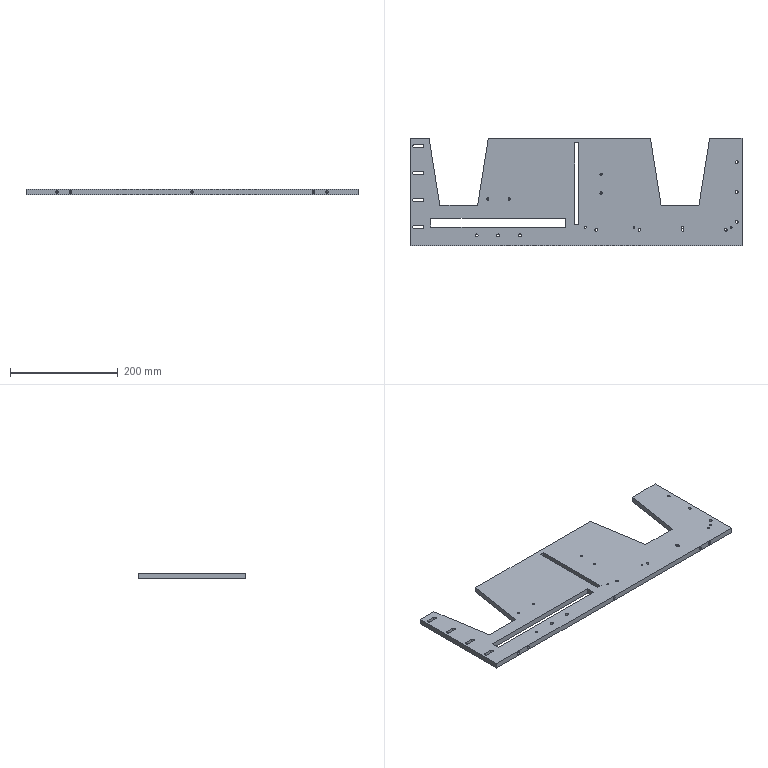Component | SolidWorks | P-SLJ-001-008-1 | 1 solid | 108 faces | box 615 x 200 x 10 mm | volume 942437 mm3 | cylinder 64 | plane 34 | cone 10 | commonest cylinder face diameters 5.5 x24 5 x18 3.3 x8 4.2 x8 10 x6 | material 45#
build123d program:
from build123d import *

# Parameters (mm, degrees)
SKETCH1_W                                            = 615
SKETCH1_H                                            = 200
EXTRUDE1_DEPTH                                       = 5
TAP_DRILL_FOR_M4X0_5_TAP1_D                          = 5.5
EXTRUDE2_DEPTH                                       = 324.506
M6_TAPPED_HOLE1_D                                    = 5
SKETCH9_W                                            = 8
SKETCH9_H                                            = 151
EXTRUDE3_DEPTH                                       = 324.506
EXTRUDE4_DEPTH                                       = 324.506
M5_TAPPED_HOLE1_2_D                                  = 4.2
HOLE_SIZE_ACCORDING_TO_TYPE_OF_HEX_SOCKE_D           = 5.5
HOLE_SIZE_ACCORDING_TO_TYPE_OF_HEX_SOCKE_CBORE_D     = 10
HOLE_SIZE_ACCORDING_TO_TYPE_OF_HEX_SOCKE_CBORE_DEPTH = 5.7
SKETCH16_W                                           = 250
SKETCH16_H                                           = 16
EXTRUDE5_DEPTH                                       = 324.506
M5_TAPPED_HOLE1_D                                    = 4.2
CHAMFER1_SIZE                                        = 2
CHAMFER1_SIZE2                                       = 5
M4_TAPPED_HOLE3_D                                    = 3.3
F_5_0_5_DIAMETER_HOLE1_D                             = 5
F_5_0_5_DIAMETER_HOLE1_DEPTH                         = 10
F_5_0_5_DIAMETER_HOLE1_TIP                           = 1.502
M6_TAPPED_HOLE2_D                                    = 5
M6_TAPPED_HOLE2_DEPTH                                = 17
M6_TAPPED_HOLE2_TIP                                  = 1.502


with BuildPart() as part:
    # Sketch1 → Extrude1 (new, symmetric)
    with BuildSketch(Plane.XY):
        Rectangle(SKETCH1_W, SKETCH1_H)
    extrude(amount=EXTRUDE1_DEPTH, both=True)

    # Tap Drill for M4X0.5 Tap1 (through all)
    with Locations(Plane.XY.offset(5)):
        with Locations((297.5, 55), (297.5, 0), (297.5, -55)):
            Hole(TAP_DRILL_FOR_M4X0_5_TAP1_D / 2)

    # Sketch5 → Extrude2 (cut, through all)
    with BuildSketch(Plane.XY.offset(5)):
        Polygon((137.904, 100), (247.5, 100), (227.702, -25), (157.702, -25), align=None)
        Polygon((-272.096, 100), (-162.5, 100), (-182.298, -25), (-252.298, -25), align=None)
    extrude(amount=-EXTRUDE2_DEPTH, mode=Mode.SUBTRACT)

    # M6 Tapped Hole1 (through all)
    with Locations(Plane.XY.offset(5)):
        with Locations((37.5, -70), (117.5, -70), (197.5, -70), (277.5, -70)):
            Hole(M6_TAPPED_HOLE1_D / 2)

    # Sketch9 → Extrude3 (cut, through all)
    with BuildSketch(Plane.XY.offset(5)):
        with Locations((1.5, 15.5)):
            Rectangle(SKETCH9_W, SKETCH9_H)
    extrude(amount=-EXTRUDE3_DEPTH, mode=Mode.SUBTRACT)

    # Sketch10 → Extrude4 (cut, through all)
    with BuildSketch(Plane.XY.offset(5)):
        with BuildLine():
            Line((-300, 87.75), (-285, 87.75))
            ThreePointArc((-285, 87.75), (-282.25, 85), (-285, 82.25))
            Line((-285, 82.25), (-300, 82.25))
            ThreePointArc((-300, 82.25), (-302.75, 85), (-300, 87.75))
        make_face()
        with BuildLine():
            Line((-300, 37.75), (-285, 37.75))
            ThreePointArc((-285, 37.75), (-282.25, 35), (-285, 32.25))
            Line((-285, 32.25), (-300, 32.25))
            ThreePointArc((-300, 32.25), (-302.75, 35), (-300, 37.75))
        make_face()
        with BuildLine():
            Line((-300, -12.25), (-285, -12.25))
            ThreePointArc((-285, -12.25), (-282.25, -15), (-285, -17.75))
            Line((-285, -17.75), (-300, -17.75))
            ThreePointArc((-300, -17.75), (-302.75, -15), (-300, -12.25))
        make_face()
        with BuildLine():
            Line((-300, -62.25), (-285, -62.25))
            ThreePointArc((-285, -62.25), (-282.25, -65), (-285, -67.75))
            Line((-285, -67.75), (-300, -67.75))
            ThreePointArc((-300, -67.75), (-302.75, -65), (-300, -62.25))
        make_face()
    extrude(amount=-EXTRUDE4_DEPTH, mode=Mode.SUBTRACT)

    # M5 Tapped Hole1_2 (through all)
    with Locations(Plane.XY.offset(5)):
        with Locations((-163.5, -13), (-123.5, -13)):
            Hole(M5_TAPPED_HOLE1_2_D / 2)

    # Hole Size_according to_Type of Hex Socke (through all)
    with Locations(Plane(origin=(0, 0, -5), x_dir=(-1, 0, 0), z_dir=(0, 0, -1))):
        with Locations((184, -80.5), (144, -80.5), (104, -80.5)):
            CounterBoreHole(HOLE_SIZE_ACCORDING_TO_TYPE_OF_HEX_SOCKE_D / 2, HOLE_SIZE_ACCORDING_TO_TYPE_OF_HEX_SOCKE_CBORE_D / 2, HOLE_SIZE_ACCORDING_TO_TYPE_OF_HEX_SOCKE_CBORE_DEPTH)

    # Sketch16 → Extrude5 (cut, through all)
    with BuildSketch(Plane.XY.offset(5)):
        with Locations((-144, -57)):
            Rectangle(SKETCH16_W, SKETCH16_H)
    extrude(amount=-EXTRUDE5_DEPTH, mode=Mode.SUBTRACT)

    # M5 Tapped Hole1 (through all)
    with Locations(Plane.XY.offset(5)):
        with Locations((46.5, 33), (46.5, -2)):
            Hole(M5_TAPPED_HOLE1_D / 2)

    # Chamfer1
    chamfer1_edges = [part.edges().sort_by_distance(p)[0] for p in [
        (-144, -65, -5),
    ]]
    chamfer1_side = [part.faces().sort_by_distance(p)[0] for p in [
        (-144, -65, 0),
    ]]
    chamfer(chamfer1_edges, length=CHAMFER1_SIZE, length2=CHAMFER1_SIZE2, reference=chamfer1_side[0])

    # M4 Tapped Hole3 (through all)
    with Locations(Plane(origin=(0, 0, -5), x_dir=(-1, 0, 0), z_dir=(0, 0, -1))):
        with Locations((-287.5, -65.5), (-197.5, -65.5), (-107.5, -65.5), (-17.5, -65.5)):
            Hole(M4_TAPPED_HOLE3_D / 2)

    # 5.0 _5_ Diameter Hole1
    with Locations(Plane(origin=(0, -100, 0), x_dir=(-1, 0, 0), z_dir=(0, -1, 0))):
        with Locations((225, 0), (-225, 0)):
            Hole(F_5_0_5_DIAMETER_HOLE1_D / 2, depth=F_5_0_5_DIAMETER_HOLE1_DEPTH)
            with Locations((0, 0, -(F_5_0_5_DIAMETER_HOLE1_DEPTH + F_5_0_5_DIAMETER_HOLE1_TIP / 2))):  # 118° drill point
                Cone(0, F_5_0_5_DIAMETER_HOLE1_D / 2, F_5_0_5_DIAMETER_HOLE1_TIP, mode=Mode.SUBTRACT)

    # M6 Tapped Hole2
    with Locations(Plane(origin=(0, -100, 0), x_dir=(-1, 0, 0), z_dir=(0, -1, 0))):
        with Locations((250, 0), (0, 0), (-250, 0)):
            Hole(M6_TAPPED_HOLE2_D / 2, depth=M6_TAPPED_HOLE2_DEPTH)
            with Locations((0, 0, -(M6_TAPPED_HOLE2_DEPTH + M6_TAPPED_HOLE2_TIP / 2))):  # 118° drill point
                Cone(0, M6_TAPPED_HOLE2_D / 2, M6_TAPPED_HOLE2_TIP, mode=Mode.SUBTRACT)


solid = part.part

# Placed as in the assembly
solid = solid.moved(Location((-76, 0, 1230.634), (0, 0, 0)))